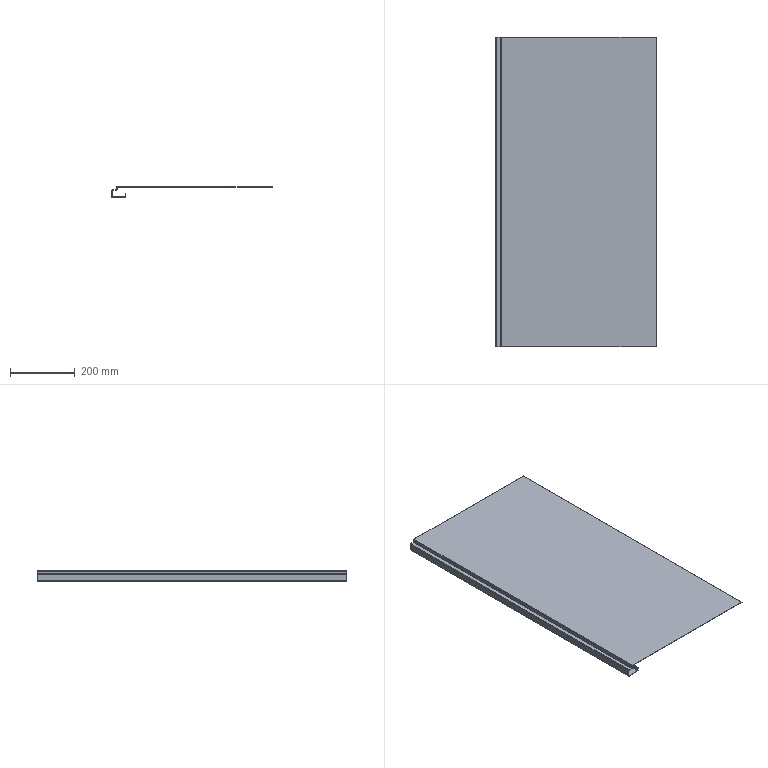Component | SolidWorks | Shelf-1 | 1 solid | 46 faces | volume 663855 mm3 | plane 36 | cylinder 10 | commonest cylinder face diameters 4.4 x5 2 x5